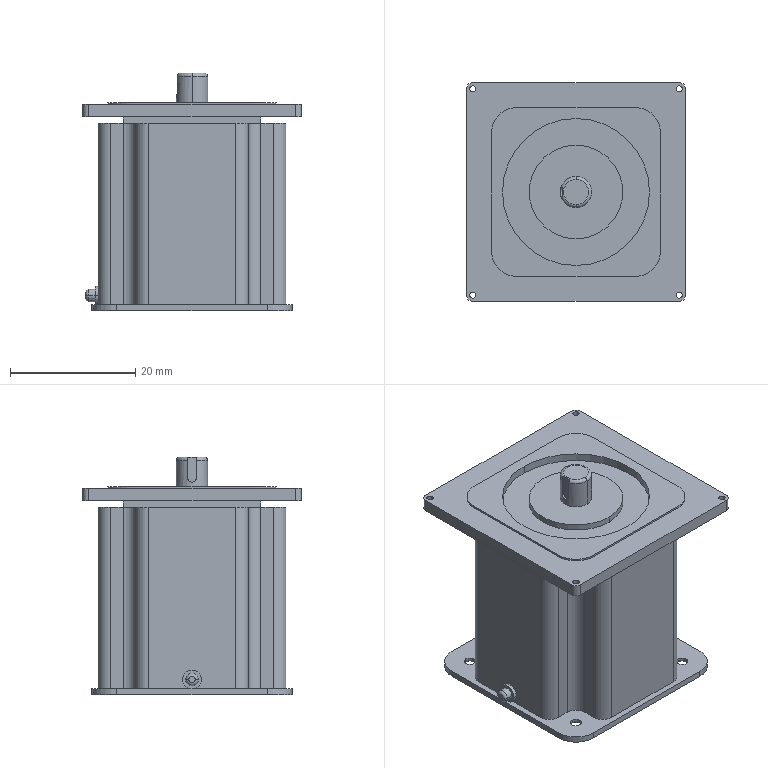Component | SolidWorks | GMotor-1 | 1 solid | 113 faces | volume 25677 mm3 | cylinder 52 | plane 49 | cone 8 | torus 4 | commonest cylinder face diameters 4 x12 1.778 x8 1 x8 8 x8 2 x6 3 x3 23.5 x2 15 x2